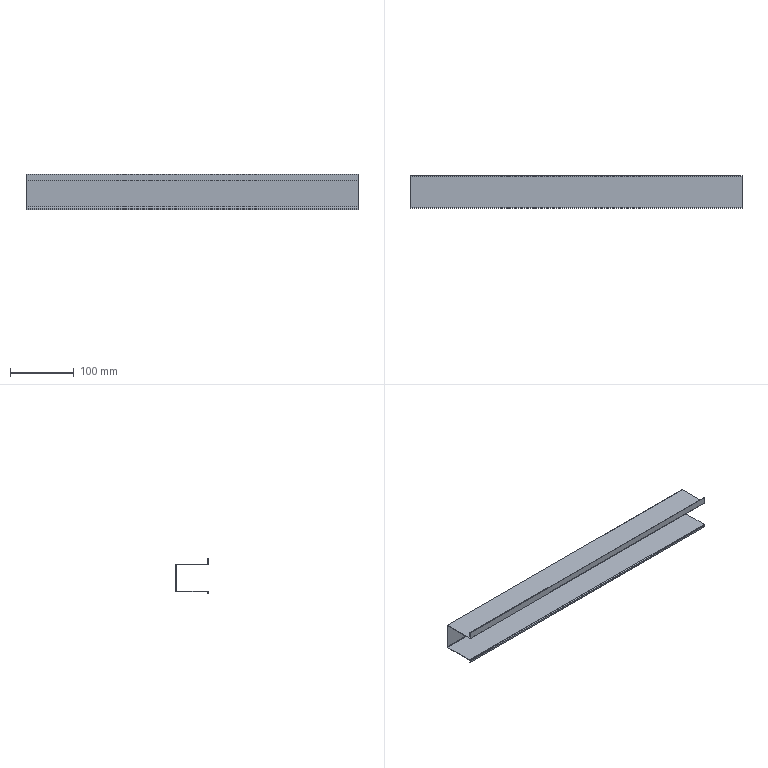Component | SolidWorks | ConnectingFlange-3 | 2 solids | 26 faces | box 520 x 50.74 x 56.23 mm | volume 59197 mm3 | plane 22 | cylinder 4 | commonest cylinder face diameters 2.946 x2 1.473 x2
STEP:
#1=CARTESIAN_POINT('',(-10.906,0.8454,1.916));
#2=VERTEX_POINT('',#1);
#3=CARTESIAN_POINT('',(-10.906,0.8454,1.945));
#4=VERTEX_POINT('',#3);
#5=CARTESIAN_POINT('',(-10.906,0.8454,1.916));
#6=DIRECTION('',(0.,-0.,1.));
#7=VECTOR('',#6,39.37);
#8=LINE('',#5,#7);
#9=EDGE_CURVE('',#2,#4,#8,.T.);
#10=ORIENTED_EDGE('',*,*,#9,.T.);
#11=CARTESIAN_POINT('',(-10.906,2.727,1.945));
#12=VERTEX_POINT('',#11);
#13=CARTESIAN_POINT('',(-10.906,2.756,1.945));
#14=DIRECTION('',(-0.,1.,0.));
#15=VECTOR('',#14,39.37);
#16=LINE('',#13,#15);
#17=EDGE_CURVE('',#4,#12,#16,.T.);
#18=ORIENTED_EDGE('',*,*,#17,.T.);
#19=CARTESIAN_POINT('',(-10.906,2.727,1.916));
#20=VERTEX_POINT('',#19);
#21=CARTESIAN_POINT('',(-10.906,2.727,1.916));
#22=DIRECTION('',(0.,0.,-1.));
#23=VECTOR('',#22,39.37);
#24=LINE('',#21,#23);
#25=EDGE_CURVE('',#12,#20,#24,.T.);
#26=ORIENTED_EDGE('',*,*,#25,.T.);
#27=CARTESIAN_POINT('',(-10.906,0.7874,1.916));
#28=DIRECTION('',(-0.,1.,0.));
#29=VECTOR('',#28,39.37);
#30=LINE('',#27,#29);
#31=EDGE_CURVE('',#2,#20,#30,.T.);
#32=ORIENTED_EDGE('',*,*,#31,.F.);
#33=EDGE_LOOP('',(#10,#18,#26,#32));
#34=FACE_OUTER_BOUND('',#33,.T.);
#35=CARTESIAN_POINT('',(-10.906,2.756,1.916));
#36=DIRECTION('',(1.,-0.,0.));
#37=DIRECTION('',(0.,0.,-1.));
#38=AXIS2_PLACEMENT_3D('',#35,#36,#37);
#39=PLANE('',#38);
#40=ADVANCED_FACE('',(#34),#39,.F.);
#41=CARTESIAN_POINT('',(9.567,2.727,1.916));
#42=VERTEX_POINT('',#41);
#43=CARTESIAN_POINT('',(-10.906,2.727,1.916));
#44=DIRECTION('',(-1.,0.,-0.));
#45=VECTOR('',#44,39.37);
#46=LINE('',#43,#45);
#47=EDGE_CURVE('',#42,#20,#46,.T.);
#48=ORIENTED_EDGE('',*,*,#47,.F.);
#49=CARTESIAN_POINT('',(9.567,0.8454,1.916));
#50=VERTEX_POINT('',#49);
#51=CARTESIAN_POINT('',(9.567,0.7874,1.916));
#52=DIRECTION('',(0.,-1.,-0.));
#53=VECTOR('',#52,39.37);
#54=LINE('',#51,#53);
#55=EDGE_CURVE('',#42,#50,#54,.T.);
#56=ORIENTED_EDGE('',*,*,#55,.T.);
#57=CARTESIAN_POINT('',(-10.906,0.8454,1.916));
#58=DIRECTION('',(1.,-0.,-0.));
#59=VECTOR('',#58,39.37);
#60=LINE('',#57,#59);
#61=EDGE_CURVE('',#2,#50,#60,.T.);
#62=ORIENTED_EDGE('',*,*,#61,.F.);
#63=ORIENTED_EDGE('',*,*,#31,.T.);
#64=EDGE_LOOP('',(#48,#56,#62,#63));
#65=FACE_OUTER_BOUND('',#64,.T.);
#66=CARTESIAN_POINT('',(0.,0.7874,1.916));
#67=DIRECTION('',(-0.,-0.,1.));
#68=DIRECTION('',(-0.,1.,0.));
#69=AXIS2_PLACEMENT_3D('',#66,#67,#68);
#70=PLANE('',#69);
#71=ADVANCED_FACE('',(#65),#70,.F.);
#72=CARTESIAN_POINT('',(9.567,2.727,1.945));
#73=VERTEX_POINT('',#72);
#74=CARTESIAN_POINT('',(9.567,0.8454,1.945));
#75=VERTEX_POINT('',#74);
#76=CARTESIAN_POINT('',(9.567,0.7874,1.945));
#77=DIRECTION('',(0.,-1.,-0.));
#78=VECTOR('',#77,39.37);
#79=LINE('',#76,#78);
#80=EDGE_CURVE('',#73,#75,#79,.T.);
#81=ORIENTED_EDGE('',*,*,#80,.F.);
#82=CARTESIAN_POINT('',(-10.906,2.727,1.945));
#83=DIRECTION('',(1.,-0.,0.));
#84=VECTOR('',#83,39.37);
#85=LINE('',#82,#84);
#86=EDGE_CURVE('',#12,#73,#85,.T.);
#87=ORIENTED_EDGE('',*,*,#86,.F.);
#88=ORIENTED_EDGE('',*,*,#17,.F.);
#89=CARTESIAN_POINT('',(-10.906,0.8454,1.945));
#90=DIRECTION('',(1.,-0.,-0.));
#91=VECTOR('',#90,39.37);
#92=LINE('',#89,#91);
#93=EDGE_CURVE('',#4,#75,#92,.T.);
#94=ORIENTED_EDGE('',*,*,#93,.T.);
#95=EDGE_LOOP('',(#81,#87,#88,#94));
#96=FACE_OUTER_BOUND('',#95,.T.);
#97=CARTESIAN_POINT('',(0.,0.7874,1.945));
#98=DIRECTION('',(-0.,-0.,1.));
#99=DIRECTION('',(-0.,1.,0.));
#100=AXIS2_PLACEMENT_3D('',#97,#98,#99);
#101=PLANE('',#100);
#102=ADVANCED_FACE('',(#96),#101,.T.);
#103=CARTESIAN_POINT('',(-10.906,2.785,3.579));
#104=VERTEX_POINT('',#103);
#105=CARTESIAN_POINT('',(9.567,2.785,3.579));
#106=VERTEX_POINT('',#105);
#107=CARTESIAN_POINT('',(-10.906,2.785,3.579));
#108=DIRECTION('',(1.,-0.,-0.));
#109=VECTOR('',#108,39.37);
#110=LINE('',#107,#109);
#111=EDGE_CURVE('',#104,#106,#110,.T.);
#112=ORIENTED_EDGE('',*,*,#111,.T.);
#113=CARTESIAN_POINT('',(9.567,2.785,1.974));
#114=VERTEX_POINT('',#113);
#115=CARTESIAN_POINT('',(9.567,2.785,-19.895));
#116=DIRECTION('',(-0.,0.,-1.));
#117=VECTOR('',#116,39.37);
#118=LINE('',#115,#117);
#119=EDGE_CURVE('',#106,#114,#118,.T.);
#120=ORIENTED_EDGE('',*,*,#119,.T.);
#121=CARTESIAN_POINT('',(-10.906,2.785,1.974));
#122=VERTEX_POINT('',#121);
#123=CARTESIAN_POINT('',(10.906,2.785,1.974));
#124=DIRECTION('',(-1.,0.,0.));
#125=VECTOR('',#124,39.37);
#126=LINE('',#123,#125);
#127=EDGE_CURVE('',#114,#122,#126,.T.);
#128=ORIENTED_EDGE('',*,*,#127,.T.);
#129=CARTESIAN_POINT('',(-10.906,2.785,-19.895));
#130=DIRECTION('',(0.,-0.,1.));
#131=VECTOR('',#130,39.37);
#132=LINE('',#129,#131);
#133=EDGE_CURVE('',#122,#104,#132,.T.);
#134=ORIENTED_EDGE('',*,*,#133,.T.);
#135=EDGE_LOOP('',(#112,#120,#128,#134));
#136=FACE_OUTER_BOUND('',#135,.T.);
#137=CARTESIAN_POINT('',(-10.906,2.785,-19.895));
#138=DIRECTION('',(-0.,-1.,-0.));
#139=DIRECTION('',(1.,-0.,-0.));
#140=AXIS2_PLACEMENT_3D('',#137,#138,#139);
#141=PLANE('',#140);
#142=ADVANCED_FACE('',(#136),#141,.F.);
#143=CARTESIAN_POINT('',(9.567,2.756,3.579));
#144=VERTEX_POINT('',#143);
#145=CARTESIAN_POINT('',(9.567,2.756,1.974));
#146=VERTEX_POINT('',#145);
#147=CARTESIAN_POINT('',(9.567,2.756,-19.895));
#148=DIRECTION('',(-0.,0.,-1.));
#149=VECTOR('',#148,39.37);
#150=LINE('',#147,#149);
#151=EDGE_CURVE('',#144,#146,#150,.T.);
#152=ORIENTED_EDGE('',*,*,#151,.F.);
#153=CARTESIAN_POINT('',(-10.906,2.756,3.579));
#154=VERTEX_POINT('',#153);
#155=CARTESIAN_POINT('',(-10.906,2.756,3.579));
#156=DIRECTION('',(1.,-0.,-0.));
#157=VECTOR('',#156,39.37);
#158=LINE('',#155,#157);
#159=EDGE_CURVE('',#154,#144,#158,.T.);
#160=ORIENTED_EDGE('',*,*,#159,.F.);
#161=CARTESIAN_POINT('',(-10.906,2.756,1.974));
#162=VERTEX_POINT('',#161);
#163=CARTESIAN_POINT('',(-10.906,2.756,-19.895));
#164=DIRECTION('',(0.,-0.,1.));
#165=VECTOR('',#164,39.37);
#166=LINE('',#163,#165);
#167=EDGE_CURVE('',#162,#154,#166,.T.);
#168=ORIENTED_EDGE('',*,*,#167,.F.);
#169=CARTESIAN_POINT('',(10.906,2.756,1.974));
#170=DIRECTION('',(-1.,0.,0.));
#171=VECTOR('',#170,39.37);
#172=LINE('',#169,#171);
#173=EDGE_CURVE('',#146,#162,#172,.T.);
#174=ORIENTED_EDGE('',*,*,#173,.F.);
#175=EDGE_LOOP('',(#152,#160,#168,#174));
#176=FACE_OUTER_BOUND('',#175,.T.);
#177=CARTESIAN_POINT('',(-10.906,2.756,-19.895));
#178=DIRECTION('',(-0.,-1.,-0.));
#179=DIRECTION('',(1.,-0.,-0.));
#180=AXIS2_PLACEMENT_3D('',#177,#178,#179);
#181=PLANE('',#180);
#182=ADVANCED_FACE('',(#176),#181,.T.);
#183=CARTESIAN_POINT('',(-10.906,2.756,1.974));
#184=DIRECTION('',(-0.,1.,0.));
#185=VECTOR('',#184,39.37);
#186=LINE('',#183,#185);
#187=EDGE_CURVE('',#162,#122,#186,.T.);
#188=ORIENTED_EDGE('',*,*,#187,.F.);
#189=ORIENTED_EDGE('',*,*,#167,.T.);
#190=CARTESIAN_POINT('',(-10.906,2.785,3.579));
#191=DIRECTION('',(0.,-1.,-0.));
#192=VECTOR('',#191,39.37);
#193=LINE('',#190,#192);
#194=EDGE_CURVE('',#104,#154,#193,.T.);
#195=ORIENTED_EDGE('',*,*,#194,.F.);
#196=ORIENTED_EDGE('',*,*,#133,.F.);
#197=EDGE_LOOP('',(#188,#189,#195,#196));
#198=FACE_OUTER_BOUND('',#197,.T.);
#199=CARTESIAN_POINT('',(-10.906,2.785,-19.895));
#200=DIRECTION('',(-1.,-0.,-0.));
#201=DIRECTION('',(0.,-1.,-0.));
#202=AXIS2_PLACEMENT_3D('',#199,#200,#201);
#203=PLANE('',#202);
#204=ADVANCED_FACE('',(#198),#203,.T.);
#205=ORIENTED_EDGE('',*,*,#159,.T.);
#206=CARTESIAN_POINT('',(9.567,0.7874,3.579));
#207=DIRECTION('',(-0.,1.,0.));
#208=VECTOR('',#207,39.37);
#209=LINE('',#206,#208);
#210=EDGE_CURVE('',#144,#106,#209,.T.);
#211=ORIENTED_EDGE('',*,*,#210,.T.);
#212=ORIENTED_EDGE('',*,*,#111,.F.);
#213=ORIENTED_EDGE('',*,*,#194,.T.);
#214=EDGE_LOOP('',(#205,#211,#212,#213));
#215=FACE_OUTER_BOUND('',#214,.T.);
#216=CARTESIAN_POINT('',(0.,0.7874,3.579));
#217=DIRECTION('',(0.,0.,-1.));
#218=DIRECTION('',(-1.,0.,0.));
#219=AXIS2_PLACEMENT_3D('',#216,#217,#218);
#220=PLANE('',#219);
#221=ADVANCED_FACE('',(#215),#220,.F.);
#222=ORIENTED_EDGE('',*,*,#25,.F.);
#223=CARTESIAN_POINT('',(-10.906,2.727,1.974));
#224=DIRECTION('',(-1.,0.,0.));
#225=DIRECTION('',(0.,1.,-0.));
#226=AXIS2_PLACEMENT_3D('',#223,#224,#225);
#227=CIRCLE('',#226,0.029);
#228=EDGE_CURVE('',#162,#12,#227,.T.);
#229=ORIENTED_EDGE('',*,*,#228,.F.);
#230=ORIENTED_EDGE('',*,*,#187,.T.);
#231=CARTESIAN_POINT('',(-10.906,2.727,1.974));
#232=DIRECTION('',(-1.,0.,0.));
#233=DIRECTION('',(0.,1.,0.));
#234=AXIS2_PLACEMENT_3D('',#231,#232,#233);
#235=CIRCLE('',#234,0.058);
#236=EDGE_CURVE('',#122,#20,#235,.T.);
#237=ORIENTED_EDGE('',*,*,#236,.T.);
#238=EDGE_LOOP('',(#222,#229,#230,#237));
#239=FACE_OUTER_BOUND('',#238,.T.);
#240=CARTESIAN_POINT('',(-10.906,2.727,1.974));
#241=DIRECTION('',(-1.,-0.,-0.));
#242=DIRECTION('',(0.,-1.,-0.));
#243=AXIS2_PLACEMENT_3D('',#240,#241,#242);
#244=PLANE('',#243);
#245=ADVANCED_FACE('',(#239),#244,.T.);
#246=CARTESIAN_POINT('',(9.567,2.727,1.974));
#247=DIRECTION('',(1.,-0.,-0.));
#248=DIRECTION('',(0.,-1.,0.));
#249=AXIS2_PLACEMENT_3D('',#246,#247,#248);
#250=CIRCLE('',#249,0.058);
#251=EDGE_CURVE('',#42,#114,#250,.T.);
#252=ORIENTED_EDGE('',*,*,#251,.F.);
#253=ORIENTED_EDGE('',*,*,#47,.T.);
#254=ORIENTED_EDGE('',*,*,#236,.F.);
#255=ORIENTED_EDGE('',*,*,#127,.F.);
#256=EDGE_LOOP('',(#252,#253,#254,#255));
#257=FACE_OUTER_BOUND('',#256,.T.);
#258=CARTESIAN_POINT('',(10.906,2.727,1.974));
#259=DIRECTION('',(1.,-0.,-0.));
#260=DIRECTION('',(0.,0.,-1.));
#261=AXIS2_PLACEMENT_3D('',#258,#259,#260);
#262=CYLINDRICAL_SURFACE('',#261,0.058);
#263=ADVANCED_FACE('',(#257),#262,.T.);
#264=ORIENTED_EDGE('',*,*,#86,.T.);
#265=CARTESIAN_POINT('',(9.567,2.727,1.974));
#266=DIRECTION('',(1.,-0.,-0.));
#267=DIRECTION('',(0.,-1.,0.));
#268=AXIS2_PLACEMENT_3D('',#265,#266,#267);
#269=CIRCLE('',#268,0.029);
#270=EDGE_CURVE('',#73,#146,#269,.T.);
#271=ORIENTED_EDGE('',*,*,#270,.T.);
#272=ORIENTED_EDGE('',*,*,#173,.T.);
#273=ORIENTED_EDGE('',*,*,#228,.T.);
#274=EDGE_LOOP('',(#264,#271,#272,#273));
#275=FACE_OUTER_BOUND('',#274,.T.);
#276=CARTESIAN_POINT('',(10.906,2.727,1.974));
#277=DIRECTION('',(1.,-0.,-0.));
#278=DIRECTION('',(0.,0.,-1.));
#279=AXIS2_PLACEMENT_3D('',#276,#277,#278);
#280=CYLINDRICAL_SURFACE('',#279,0.029);
#281=ADVANCED_FACE('',(#275),#280,.F.);
#282=CARTESIAN_POINT('',(-10.906,0.8164,1.887));
#283=VERTEX_POINT('',#282);
#284=CARTESIAN_POINT('',(-10.906,0.8454,1.887));
#285=DIRECTION('',(-1.,0.,0.));
#286=DIRECTION('',(0.,-1.,0.));
#287=AXIS2_PLACEMENT_3D('',#284,#285,#286);
#288=CIRCLE('',#287,0.029);
#289=EDGE_CURVE('',#283,#2,#288,.T.);
#290=ORIENTED_EDGE('',*,*,#289,.F.);
#291=CARTESIAN_POINT('',(-10.906,0.7874,1.887));
#292=VERTEX_POINT('',#291);
#293=CARTESIAN_POINT('',(-10.906,0.8164,1.887));
#294=DIRECTION('',(0.,-1.,0.));
#295=VECTOR('',#294,39.37);
#296=LINE('',#293,#295);
#297=EDGE_CURVE('',#283,#292,#296,.T.);
#298=ORIENTED_EDGE('',*,*,#297,.T.);
#299=CARTESIAN_POINT('',(-10.906,0.8454,1.887));
#300=DIRECTION('',(-1.,0.,0.));
#301=DIRECTION('',(0.,-1.,0.));
#302=AXIS2_PLACEMENT_3D('',#299,#300,#301);
#303=CIRCLE('',#302,0.058);
#304=EDGE_CURVE('',#292,#4,#303,.T.);
#305=ORIENTED_EDGE('',*,*,#304,.T.);
#306=ORIENTED_EDGE('',*,*,#9,.F.);
#307=EDGE_LOOP('',(#290,#298,#305,#306));
#308=FACE_OUTER_BOUND('',#307,.T.);
#309=CARTESIAN_POINT('',(-10.906,0.8454,1.887));
#310=DIRECTION('',(1.,-0.,-0.));
#311=DIRECTION('',(0.,1.,0.));
#312=AXIS2_PLACEMENT_3D('',#309,#310,#311);
#313=PLANE('',#312);
#314=ADVANCED_FACE('',(#308),#313,.F.);
#315=CARTESIAN_POINT('',(9.567,0.7874,1.887));
#316=VERTEX_POINT('',#315);
#317=CARTESIAN_POINT('',(9.567,0.8454,1.887));
#318=DIRECTION('',(1.,-0.,-0.));
#319=DIRECTION('',(0.,-1.,-0.));
#320=AXIS2_PLACEMENT_3D('',#317,#318,#319);
#321=CIRCLE('',#320,0.058);
#322=EDGE_CURVE('',#75,#316,#321,.T.);
#323=ORIENTED_EDGE('',*,*,#322,.F.);
#324=ORIENTED_EDGE('',*,*,#93,.F.);
#325=ORIENTED_EDGE('',*,*,#304,.F.);
#326=CARTESIAN_POINT('',(10.906,0.7874,1.887));
#327=DIRECTION('',(1.,-0.,0.));
#328=VECTOR('',#327,39.37);
#329=LINE('',#326,#328);
#330=EDGE_CURVE('',#292,#316,#329,.T.);
#331=ORIENTED_EDGE('',*,*,#330,.T.);
#332=EDGE_LOOP('',(#323,#324,#325,#331));
#333=FACE_OUTER_BOUND('',#332,.T.);
#334=CARTESIAN_POINT('',(-10.906,0.8454,1.887));
#335=DIRECTION('',(-1.,0.,0.));
#336=DIRECTION('',(0.,-1.,0.));
#337=AXIS2_PLACEMENT_3D('',#334,#335,#336);
#338=CYLINDRICAL_SURFACE('',#337,0.058);
#339=ADVANCED_FACE('',(#333),#338,.T.);
#340=ORIENTED_EDGE('',*,*,#61,.T.);
#341=CARTESIAN_POINT('',(9.567,0.8164,1.887));
#342=VERTEX_POINT('',#341);
#343=CARTESIAN_POINT('',(9.567,0.8454,1.887));
#344=DIRECTION('',(1.,-0.,-0.));
#345=DIRECTION('',(0.,-1.,-0.));
#346=AXIS2_PLACEMENT_3D('',#343,#344,#345);
#347=CIRCLE('',#346,0.029);
#348=EDGE_CURVE('',#50,#342,#347,.T.);
#349=ORIENTED_EDGE('',*,*,#348,.T.);
#350=CARTESIAN_POINT('',(10.906,0.8164,1.887));
#351=DIRECTION('',(-1.,0.,-0.));
#352=VECTOR('',#351,39.37);
#353=LINE('',#350,#352);
#354=EDGE_CURVE('',#342,#283,#353,.T.);
#355=ORIENTED_EDGE('',*,*,#354,.T.);
#356=ORIENTED_EDGE('',*,*,#289,.T.);
#357=EDGE_LOOP('',(#340,#349,#355,#356));
#358=FACE_OUTER_BOUND('',#357,.T.);
#359=CARTESIAN_POINT('',(-10.906,0.8454,1.887));
#360=DIRECTION('',(-1.,0.,0.));
#361=DIRECTION('',(0.,-1.,0.));
#362=AXIS2_PLACEMENT_3D('',#359,#360,#361);
#363=CYLINDRICAL_SURFACE('',#362,0.029);
#364=ADVANCED_FACE('',(#358),#363,.F.);
#365=ORIENTED_EDGE('',*,*,#297,.F.);
#366=CARTESIAN_POINT('',(-10.906,0.8164,1.787));
#367=VERTEX_POINT('',#366);
#368=CARTESIAN_POINT('',(-10.906,0.8164,1.787));
#369=DIRECTION('',(-0.,0.,-1.));
#370=VECTOR('',#369,39.37);
#371=LINE('',#368,#370);
#372=EDGE_CURVE('',#283,#367,#371,.T.);
#373=ORIENTED_EDGE('',*,*,#372,.T.);
#374=CARTESIAN_POINT('',(-10.906,0.7874,1.787));
#375=VERTEX_POINT('',#374);
#376=CARTESIAN_POINT('',(-10.906,0.7874,1.787));
#377=DIRECTION('',(-0.,1.,0.));
#378=VECTOR('',#377,39.37);
#379=LINE('',#376,#378);
#380=EDGE_CURVE('',#375,#367,#379,.T.);
#381=ORIENTED_EDGE('',*,*,#380,.F.);
#382=CARTESIAN_POINT('',(-10.906,0.7874,0.));
#383=DIRECTION('',(-0.,0.,-1.));
#384=VECTOR('',#383,39.37);
#385=LINE('',#382,#384);
#386=EDGE_CURVE('',#292,#375,#385,.T.);
#387=ORIENTED_EDGE('',*,*,#386,.F.);
#388=EDGE_LOOP('',(#365,#373,#381,#387));
#389=FACE_OUTER_BOUND('',#388,.T.);
#390=CARTESIAN_POINT('',(-10.906,0.7874,1.787));
#391=DIRECTION('',(1.,0.,0.));
#392=DIRECTION('',(-0.,1.,0.));
#393=AXIS2_PLACEMENT_3D('',#390,#391,#392);
#394=PLANE('',#393);
#395=ADVANCED_FACE('',(#389),#394,.F.);
#396=CARTESIAN_POINT('',(9.567,0.7874,1.787));
#397=VERTEX_POINT('',#396);
#398=CARTESIAN_POINT('',(0.,0.7874,1.787));
#399=DIRECTION('',(1.,-0.,0.));
#400=VECTOR('',#399,39.37);
#401=LINE('',#398,#400);
#402=EDGE_CURVE('',#375,#397,#401,.T.);
#403=ORIENTED_EDGE('',*,*,#402,.T.);
#404=CARTESIAN_POINT('',(9.567,0.7874,-4.553));
#405=DIRECTION('',(0.,-0.,1.));
#406=VECTOR('',#405,39.37);
#407=LINE('',#404,#406);
#408=EDGE_CURVE('',#397,#316,#407,.T.);
#409=ORIENTED_EDGE('',*,*,#408,.T.);
#410=ORIENTED_EDGE('',*,*,#330,.F.);
#411=ORIENTED_EDGE('',*,*,#386,.T.);
#412=EDGE_LOOP('',(#403,#409,#410,#411));
#413=FACE_OUTER_BOUND('',#412,.T.);
#414=CARTESIAN_POINT('',(0.,0.7874,0.));
#415=DIRECTION('',(-0.,1.,0.));
#416=DIRECTION('',(-0.,0.,-1.));
#417=AXIS2_PLACEMENT_3D('',#414,#415,#416);
#418=PLANE('',#417);
#419=ADVANCED_FACE('',(#413),#418,.F.);
#420=CARTESIAN_POINT('',(9.567,0.8164,1.787));
#421=VERTEX_POINT('',#420);
#422=CARTESIAN_POINT('',(9.567,0.8164,0.));
#423=DIRECTION('',(0.,-0.,1.));
#424=VECTOR('',#423,39.37);
#425=LINE('',#422,#424);
#426=EDGE_CURVE('',#421,#342,#425,.T.);
#427=ORIENTED_EDGE('',*,*,#426,.F.);
#428=CARTESIAN_POINT('',(10.906,0.8164,1.787));
#429=DIRECTION('',(1.,-0.,0.));
#430=VECTOR('',#429,39.37);
#431=LINE('',#428,#430);
#432=EDGE_CURVE('',#367,#421,#431,.T.);
#433=ORIENTED_EDGE('',*,*,#432,.F.);
#434=ORIENTED_EDGE('',*,*,#372,.F.);
#435=ORIENTED_EDGE('',*,*,#354,.F.);
#436=EDGE_LOOP('',(#427,#433,#434,#435));
#437=FACE_OUTER_BOUND('',#436,.T.);
#438=CARTESIAN_POINT('',(0.,0.8164,0.));
#439=DIRECTION('',(-0.,1.,0.));
#440=DIRECTION('',(-0.,0.,-1.));
#441=AXIS2_PLACEMENT_3D('',#438,#439,#440);
#442=PLANE('',#441);
#443=ADVANCED_FACE('',(#437),#442,.T.);
#444=ORIENTED_EDGE('',*,*,#432,.T.);
#445=CARTESIAN_POINT('',(9.567,0.7874,1.787));
#446=DIRECTION('',(0.,-1.,-0.));
#447=VECTOR('',#446,39.37);
#448=LINE('',#445,#447);
#449=EDGE_CURVE('',#421,#397,#448,.T.);
#450=ORIENTED_EDGE('',*,*,#449,.T.);
#451=ORIENTED_EDGE('',*,*,#402,.F.);
#452=ORIENTED_EDGE('',*,*,#380,.T.);
#453=EDGE_LOOP('',(#444,#450,#451,#452));
#454=FACE_OUTER_BOUND('',#453,.T.);
#455=CARTESIAN_POINT('',(10.906,0.7874,1.787));
#456=DIRECTION('',(-0.,-0.,1.));
#457=DIRECTION('',(1.,-0.,0.));
#458=AXIS2_PLACEMENT_3D('',#455,#456,#457);
#459=PLANE('',#458);
#460=ADVANCED_FACE('',(#454),#459,.F.);
#461=ORIENTED_EDGE('',*,*,#322,.T.);
#462=ORIENTED_EDGE('',*,*,#408,.F.);
#463=ORIENTED_EDGE('',*,*,#449,.F.);
#464=ORIENTED_EDGE('',*,*,#426,.T.);
#465=ORIENTED_EDGE('',*,*,#348,.F.);
#466=ORIENTED_EDGE('',*,*,#55,.F.);
#467=ORIENTED_EDGE('',*,*,#251,.T.);
#468=ORIENTED_EDGE('',*,*,#119,.F.);
#469=ORIENTED_EDGE('',*,*,#210,.F.);
#470=ORIENTED_EDGE('',*,*,#151,.T.);
#471=ORIENTED_EDGE('',*,*,#270,.F.);
#472=ORIENTED_EDGE('',*,*,#80,.T.);
#473=EDGE_LOOP('',(#461,#462,#463,#464,#465,#466,#467,#468,#469,#470,#471,#472));
#474=FACE_OUTER_BOUND('',#473,.T.);
#475=CARTESIAN_POINT('',(9.567,0.7874,-4.553));
#476=DIRECTION('',(-1.,-0.,-0.));
#477=DIRECTION('',(0.,-1.,-0.));
#478=AXIS2_PLACEMENT_3D('',#475,#476,#477);
#479=PLANE('',#478);
#480=ADVANCED_FACE('',(#474),#479,.F.);
#481=CLOSED_SHELL('',(#40,#71,#102,#142,#182,#204,#221,#245,#263,#281,#314,#339,#364,#395,#419,#443,#460,#480));
#482=MANIFOLD_SOLID_BREP('',#481);
#483=CARTESIAN_POINT('',(9.567,0.8164,3.608));
#484=VERTEX_POINT('',#483);
#485=CARTESIAN_POINT('',(-10.906,0.8164,3.608));
#486=VERTEX_POINT('',#485);
#487=CARTESIAN_POINT('',(10.906,0.8164,3.608));
#488=DIRECTION('',(-1.,0.,0.));
#489=VECTOR('',#488,39.37);
#490=LINE('',#487,#489);
#491=EDGE_CURVE('',#484,#486,#490,.T.);
#492=ORIENTED_EDGE('',*,*,#491,.F.);
#493=CARTESIAN_POINT('',(9.567,2.756,3.608));
#494=VERTEX_POINT('',#493);
#495=CARTESIAN_POINT('',(9.567,2.756,3.608));
#496=DIRECTION('',(-0.,1.,0.));
#497=VECTOR('',#496,39.37);
#498=LINE('',#495,#497);
#499=EDGE_CURVE('',#484,#494,#498,.T.);
#500=ORIENTED_EDGE('',*,*,#499,.T.);
#501=CARTESIAN_POINT('',(-10.906,2.756,3.608));
#502=VERTEX_POINT('',#501);
#503=CARTESIAN_POINT('',(-10.906,2.756,3.608));
#504=DIRECTION('',(1.,-0.,-0.));
#505=VECTOR('',#504,39.37);
#506=LINE('',#503,#505);
#507=EDGE_CURVE('',#502,#494,#506,.T.);
#508=ORIENTED_EDGE('',*,*,#507,.F.);
#509=CARTESIAN_POINT('',(-10.906,2.756,3.608));
#510=DIRECTION('',(0.,-1.,-0.));
#511=VECTOR('',#510,39.37);
#512=LINE('',#509,#511);
#513=EDGE_CURVE('',#502,#486,#512,.T.);
#514=ORIENTED_EDGE('',*,*,#513,.T.);
#515=EDGE_LOOP('',(#492,#500,#508,#514));
#516=FACE_OUTER_BOUND('',#515,.T.);
#517=CARTESIAN_POINT('',(-10.906,2.756,3.608));
#518=DIRECTION('',(-0.,0.,-1.));
#519=DIRECTION('',(0.,-1.,-0.));
#520=AXIS2_PLACEMENT_3D('',#517,#518,#519);
#521=PLANE('',#520);
#522=ADVANCED_FACE('',(#516),#521,.F.);
#523=CARTESIAN_POINT('',(9.567,0.7874,3.579));
#524=VERTEX_POINT('',#523);
#525=CARTESIAN_POINT('',(9.567,2.756,3.579));
#526=VERTEX_POINT('',#525);
#527=CARTESIAN_POINT('',(9.567,2.756,3.579));
#528=DIRECTION('',(-0.,1.,0.));
#529=VECTOR('',#528,39.37);
#530=LINE('',#527,#529);
#531=EDGE_CURVE('',#524,#526,#530,.T.);
#532=ORIENTED_EDGE('',*,*,#531,.F.);
#533=CARTESIAN_POINT('',(-10.906,0.7874,3.579));
#534=VERTEX_POINT('',#533);
#535=CARTESIAN_POINT('',(-10.906,0.7874,3.579));
#536=DIRECTION('',(1.,-0.,-0.));
#537=VECTOR('',#536,39.37);
#538=LINE('',#535,#537);
#539=EDGE_CURVE('',#534,#524,#538,.T.);
#540=ORIENTED_EDGE('',*,*,#539,.F.);
#541=CARTESIAN_POINT('',(-10.906,2.756,3.579));
#542=VERTEX_POINT('',#541);
#543=CARTESIAN_POINT('',(-10.906,2.756,3.579));
#544=DIRECTION('',(0.,-1.,-0.));
#545=VECTOR('',#544,39.37);
#546=LINE('',#543,#545);
#547=EDGE_CURVE('',#542,#534,#546,.T.);
#548=ORIENTED_EDGE('',*,*,#547,.F.);
#549=CARTESIAN_POINT('',(-10.906,2.756,3.579));
#550=DIRECTION('',(1.,-0.,-0.));
#551=VECTOR('',#550,39.37);
#552=LINE('',#549,#551);
#553=EDGE_CURVE('',#542,#526,#552,.T.);
#554=ORIENTED_EDGE('',*,*,#553,.T.);
#555=EDGE_LOOP('',(#532,#540,#548,#554));
#556=FACE_OUTER_BOUND('',#555,.T.);
#557=CARTESIAN_POINT('',(-10.906,2.756,3.579));
#558=DIRECTION('',(-0.,0.,-1.));
#559=DIRECTION('',(0.,-1.,-0.));
#560=AXIS2_PLACEMENT_3D('',#557,#558,#559);
#561=PLANE('',#560);
#562=ADVANCED_FACE('',(#556),#561,.T.);
#563=CARTESIAN_POINT('',(-10.906,0.7874,4.001));
#564=VERTEX_POINT('',#563);
#565=CARTESIAN_POINT('',(-10.906,0.7874,3.608));
#566=DIRECTION('',(-0.,0.,-1.));
#567=VECTOR('',#566,39.37);
#568=LINE('',#565,#567);
#569=EDGE_CURVE('',#564,#534,#568,.T.);
#570=ORIENTED_EDGE('',*,*,#569,.F.);
#571=CARTESIAN_POINT('',(-10.906,0.8164,4.001));
#572=VERTEX_POINT('',#571);
#573=CARTESIAN_POINT('',(-10.906,0.7874,4.001));
#574=DIRECTION('',(-0.,1.,0.));
#575=VECTOR('',#574,39.37);
#576=LINE('',#573,#575);
#577=EDGE_CURVE('',#564,#572,#576,.T.);
#578=ORIENTED_EDGE('',*,*,#577,.T.);
#579=CARTESIAN_POINT('',(-10.906,0.8164,4.001));
#580=DIRECTION('',(-0.,0.,-1.));
#581=VECTOR('',#580,39.37);
#582=LINE('',#579,#581);
#583=EDGE_CURVE('',#572,#486,#582,.T.);
#584=ORIENTED_EDGE('',*,*,#583,.T.);
#585=ORIENTED_EDGE('',*,*,#513,.F.);
#586=CARTESIAN_POINT('',(-10.906,2.756,3.608));
#587=DIRECTION('',(-0.,0.,-1.));
#588=VECTOR('',#587,39.37);
#589=LINE('',#586,#588);
#590=EDGE_CURVE('',#502,#542,#589,.T.);
#591=ORIENTED_EDGE('',*,*,#590,.T.);
#592=ORIENTED_EDGE('',*,*,#547,.T.);
#593=EDGE_LOOP('',(#570,#578,#584,#585,#591,#592));
#594=FACE_OUTER_BOUND('',#593,.T.);
#595=CARTESIAN_POINT('',(-10.906,2.756,3.608));
#596=DIRECTION('',(-1.,-0.,-0.));
#597=DIRECTION('',(0.,-1.,-0.));
#598=AXIS2_PLACEMENT_3D('',#595,#596,#597);
#599=PLANE('',#598);
#600=ADVANCED_FACE('',(#594),#599,.T.);
#601=CARTESIAN_POINT('',(9.567,2.756,0.));
#602=DIRECTION('',(0.,-0.,1.));
#603=VECTOR('',#602,39.37);
#604=LINE('',#601,#603);
#605=EDGE_CURVE('',#526,#494,#604,.T.);
#606=ORIENTED_EDGE('',*,*,#605,.F.);
#607=ORIENTED_EDGE('',*,*,#553,.F.);
#608=ORIENTED_EDGE('',*,*,#590,.F.);
#609=ORIENTED_EDGE('',*,*,#507,.T.);
#610=EDGE_LOOP('',(#606,#607,#608,#609));
#611=FACE_OUTER_BOUND('',#610,.T.);
#612=CARTESIAN_POINT('',(0.,2.756,0.));
#613=DIRECTION('',(0.,1.,0.));
#614=DIRECTION('',(-1.,0.,0.));
#615=AXIS2_PLACEMENT_3D('',#612,#613,#614);
#616=PLANE('',#615);
#617=ADVANCED_FACE('',(#611),#616,.T.);
#618=ORIENTED_EDGE('',*,*,#539,.T.);
#619=CARTESIAN_POINT('',(9.567,0.7874,4.001));
#620=VERTEX_POINT('',#619);
#621=CARTESIAN_POINT('',(9.567,0.7874,-4.553));
#622=DIRECTION('',(0.,-0.,1.));
#623=VECTOR('',#622,39.37);
#624=LINE('',#621,#623);
#625=EDGE_CURVE('',#524,#620,#624,.T.);
#626=ORIENTED_EDGE('',*,*,#625,.T.);
#627=CARTESIAN_POINT('',(10.906,0.7874,4.001));
#628=DIRECTION('',(-1.,0.,0.));
#629=VECTOR('',#628,39.37);
#630=LINE('',#627,#629);
#631=EDGE_CURVE('',#620,#564,#630,.T.);
#632=ORIENTED_EDGE('',*,*,#631,.T.);
#633=ORIENTED_EDGE('',*,*,#569,.T.);
#634=EDGE_LOOP('',(#618,#626,#632,#633));
#635=FACE_OUTER_BOUND('',#634,.T.);
#636=CARTESIAN_POINT('',(0.,0.7874,0.));
#637=DIRECTION('',(0.,1.,0.));
#638=DIRECTION('',(-1.,0.,0.));
#639=AXIS2_PLACEMENT_3D('',#636,#637,#638);
#640=PLANE('',#639);
#641=ADVANCED_FACE('',(#635),#640,.F.);
#642=CARTESIAN_POINT('',(9.567,0.8164,4.001));
#643=VERTEX_POINT('',#642);
#644=CARTESIAN_POINT('',(10.906,0.8164,4.001));
#645=DIRECTION('',(-1.,0.,0.));
#646=VECTOR('',#645,39.37);
#647=LINE('',#644,#646);
#648=EDGE_CURVE('',#643,#572,#647,.T.);
#649=ORIENTED_EDGE('',*,*,#648,.F.);
#650=CARTESIAN_POINT('',(9.567,0.8164,4.001));
#651=DIRECTION('',(-0.,0.,-1.));
#652=VECTOR('',#651,39.37);
#653=LINE('',#650,#652);
#654=EDGE_CURVE('',#643,#484,#653,.T.);
#655=ORIENTED_EDGE('',*,*,#654,.T.);
#656=ORIENTED_EDGE('',*,*,#491,.T.);
#657=ORIENTED_EDGE('',*,*,#583,.F.);
#658=EDGE_LOOP('',(#649,#655,#656,#657));
#659=FACE_OUTER_BOUND('',#658,.T.);
#660=CARTESIAN_POINT('',(10.906,0.8164,4.001));
#661=DIRECTION('',(-0.,-1.,-0.));
#662=DIRECTION('',(1.,-0.,-0.));
#663=AXIS2_PLACEMENT_3D('',#660,#661,#662);
#664=PLANE('',#663);
#665=ADVANCED_FACE('',(#659),#664,.F.);
#666=ORIENTED_EDGE('',*,*,#631,.F.);
#667=CARTESIAN_POINT('',(9.567,0.7874,4.001));
#668=DIRECTION('',(-0.,1.,0.));
#669=VECTOR('',#668,39.37);
#670=LINE('',#667,#669);
#671=EDGE_CURVE('',#620,#643,#670,.T.);
#672=ORIENTED_EDGE('',*,*,#671,.T.);
#673=ORIENTED_EDGE('',*,*,#648,.T.);
#674=ORIENTED_EDGE('',*,*,#577,.F.);
#675=EDGE_LOOP('',(#666,#672,#673,#674));
#676=FACE_OUTER_BOUND('',#675,.T.);
#677=CARTESIAN_POINT('',(0.,0.7874,4.001));
#678=DIRECTION('',(0.,0.,-1.));
#679=DIRECTION('',(1.,-0.,-0.));
#680=AXIS2_PLACEMENT_3D('',#677,#678,#679);
#681=PLANE('',#680);
#682=ADVANCED_FACE('',(#676),#681,.F.);
#683=ORIENTED_EDGE('',*,*,#531,.T.);
#684=ORIENTED_EDGE('',*,*,#605,.T.);
#685=ORIENTED_EDGE('',*,*,#499,.F.);
#686=ORIENTED_EDGE('',*,*,#654,.F.);
#687=ORIENTED_EDGE('',*,*,#671,.F.);
#688=ORIENTED_EDGE('',*,*,#625,.F.);
#689=EDGE_LOOP('',(#683,#684,#685,#686,#687,#688));
#690=FACE_OUTER_BOUND('',#689,.T.);
#691=CARTESIAN_POINT('',(9.567,0.7874,-4.553));
#692=DIRECTION('',(-1.,-0.,-0.));
#693=DIRECTION('',(0.,-1.,-0.));
#694=AXIS2_PLACEMENT_3D('',#691,#692,#693);
#695=PLANE('',#694);
#696=ADVANCED_FACE('',(#690),#695,.F.);
#697=CLOSED_SHELL('',(#522,#562,#600,#617,#641,#665,#682,#696));
#698=MANIFOLD_SOLID_BREP('',#697);
#699=CARTESIAN_POINT('',(0.,0.,0.));
#700=DIRECTION('',(0.,0.,1.));
#701=DIRECTION('',(1.,0.,0.));
#702=AXIS2_PLACEMENT_3D('',#699,#700,#701);
#703=(LENGTH_UNIT()NAMED_UNIT(*)SI_UNIT($,.METRE.));
#704=LENGTH_MEASURE_WITH_UNIT(LENGTH_MEASURE(0.0254),#703);
#705=DIMENSIONAL_EXPONENTS(1.,0.,0.,0.,0.,0.,0.);
#706=(CONVERSION_BASED_UNIT('',#704)LENGTH_UNIT()NAMED_UNIT(#705));
#707=UNCERTAINTY_MEASURE_WITH_UNIT(LENGTH_MEASURE(0.00001),#706,'','');
#708=(NAMED_UNIT(*)PLANE_ANGLE_UNIT()SI_UNIT($,.RADIAN.));
#709=(NAMED_UNIT(*)SI_UNIT($,.STERADIAN.)SOLID_ANGLE_UNIT());
#710=(GEOMETRIC_REPRESENTATION_CONTEXT(3)GLOBAL_UNCERTAINTY_ASSIGNED_CONTEXT((#707))GLOBAL_UNIT_ASSIGNED_CONTEXT((#706,#708,#709))REPRESENTATION_CONTEXT('',''));
#711=ADVANCED_BREP_SHAPE_REPRESENTATION('',(#482,#698,#702),#710);
#712=COLOUR_RGB('',0.7922,0.8196,0.9333);
#713=FILL_AREA_STYLE_COLOUR('',#712);
#714=FILL_AREA_STYLE('',(#713));
#715=SURFACE_STYLE_FILL_AREA(#714);
#716=SURFACE_SIDE_STYLE('',(#715));
#717=SURFACE_STYLE_USAGE(.BOTH.,#716);
#718=PRESENTATION_STYLE_ASSIGNMENT((#717));
#719=STYLED_ITEM('',(#718),#482);
#720=(LENGTH_UNIT()NAMED_UNIT(*)SI_UNIT($,.METRE.));
#721=LENGTH_MEASURE_WITH_UNIT(LENGTH_MEASURE(0.0254),#720);
#722=DIMENSIONAL_EXPONENTS(1.,0.,0.,0.,0.,0.,0.);
#723=(CONVERSION_BASED_UNIT('',#721)LENGTH_UNIT()NAMED_UNIT(#722));
#724=UNCERTAINTY_MEASURE_WITH_UNIT(LENGTH_MEASURE(0.00001),#723,'','');
#725=(NAMED_UNIT(*)PLANE_ANGLE_UNIT()SI_UNIT($,.RADIAN.));
#726=(NAMED_UNIT(*)SI_UNIT($,.STERADIAN.)SOLID_ANGLE_UNIT());
#727=(GEOMETRIC_REPRESENTATION_CONTEXT(3)GLOBAL_UNCERTAINTY_ASSIGNED_CONTEXT((#724))GLOBAL_UNIT_ASSIGNED_CONTEXT((#723,#725,#726))REPRESENTATION_CONTEXT('',''));
#728=MECHANICAL_DESIGN_GEOMETRIC_PRESENTATION_REPRESENTATION('',(#719),#727);
#729=PRESENTATION_LAYER_ASSIGNMENT('','',(#719));
#730=COLOUR_RGB('',0.7922,0.8196,0.9333);
#731=FILL_AREA_STYLE_COLOUR('',#730);
#732=FILL_AREA_STYLE('',(#731));
#733=SURFACE_STYLE_FILL_AREA(#732);
#734=SURFACE_SIDE_STYLE('',(#733));
#735=SURFACE_STYLE_USAGE(.BOTH.,#734);
#736=PRESENTATION_STYLE_ASSIGNMENT((#735));
#737=STYLED_ITEM('',(#736),#698);
#738=(LENGTH_UNIT()NAMED_UNIT(*)SI_UNIT($,.METRE.));
#739=LENGTH_MEASURE_WITH_UNIT(LENGTH_MEASURE(0.0254),#738);
#740=DIMENSIONAL_EXPONENTS(1.,0.,0.,0.,0.,0.,0.);
#741=(CONVERSION_BASED_UNIT('',#739)LENGTH_UNIT()NAMED_UNIT(#740));
#742=UNCERTAINTY_MEASURE_WITH_UNIT(LENGTH_MEASURE(0.00001),#741,'','');
#743=(NAMED_UNIT(*)PLANE_ANGLE_UNIT()SI_UNIT($,.RADIAN.));
#744=(NAMED_UNIT(*)SI_UNIT($,.STERADIAN.)SOLID_ANGLE_UNIT());
#745=(GEOMETRIC_REPRESENTATION_CONTEXT(3)GLOBAL_UNCERTAINTY_ASSIGNED_CONTEXT((#742))GLOBAL_UNIT_ASSIGNED_CONTEXT((#741,#743,#744))REPRESENTATION_CONTEXT('',''));
#746=MECHANICAL_DESIGN_GEOMETRIC_PRESENTATION_REPRESENTATION('',(#737),#745);
#747=PRESENTATION_LAYER_ASSIGNMENT('','',(#737));